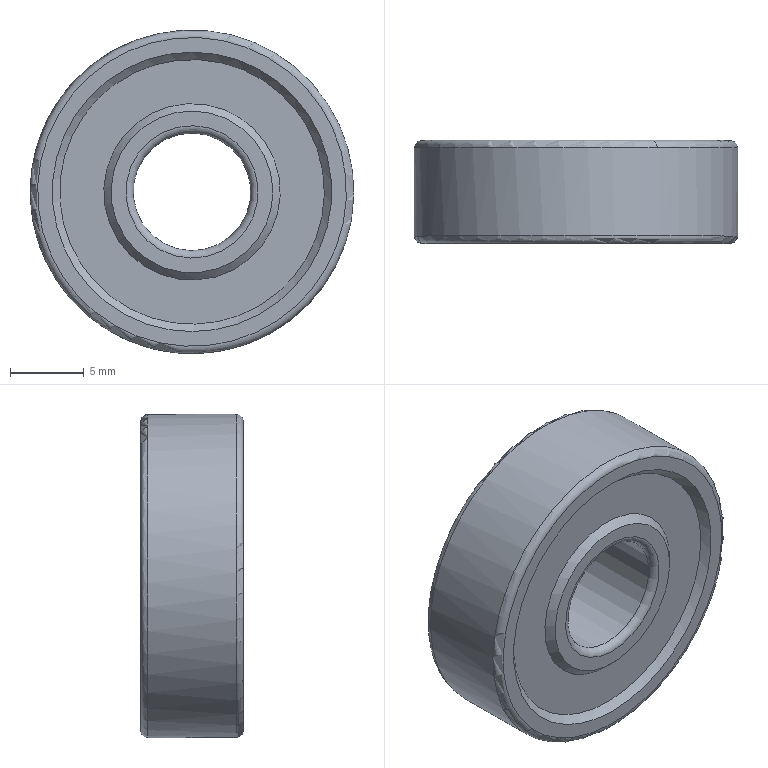Component | NX | BEARINGS | 1 solid | 16 faces | box 22 x 7 x 22 mm | volume 2134 mm3 | plane 6 | torus 4 | cone 4 | cylinder 2 | commonest cylinder face diameters 22 x1 8 x1
STEP:
#1=CARTESIAN_POINT('',(0.,0.,0.));
#2=DIRECTION('',(0.,0.,1.));
#3=DIRECTION('',(1.,0.,0.));
#4=AXIS2_PLACEMENT_3D('',#1,#2,#3);
#5=CARTESIAN_POINT('',(-426.878,103.5,-66.508));
#6=VERTEX_POINT('',#5);
#7=CARTESIAN_POINT('',(-422.274,103.5,-63.5));
#8=DIRECTION('',(0.,-1.,0.));
#9=DIRECTION('',(-0.8372,0.,-0.5469));
#10=AXIS2_PLACEMENT_3D('',#7,#8,#9);
#11=CIRCLE('',#10,5.5);
#12=CARTESIAN_POINT('',(-422.274,103.5,-63.5));
#13=DIRECTION('',(0.,-1.,0.));
#14=DIRECTION('',(-0.8372,0.,-0.5469));
#15=AXIS2_PLACEMENT_3D('',#12,#13,#14);
#16=PLANE('',#15);
#17=CARTESIAN_POINT('',(0.,0.));
#18=DIRECTION('',(1.,-0.));
#19=AXIS2_PLACEMENT_2D('',#17,#18);
#20=CIRCLE('',#19,5.5);
#21=(GEOMETRIC_REPRESENTATION_CONTEXT(2)PARAMETRIC_REPRESENTATION_CONTEXT()REPRESENTATION_CONTEXT('',''));
#22=DEFINITIONAL_REPRESENTATION('',(#20),#21);
#23=PCURVE('',#16,#22);
#24=CARTESIAN_POINT('',(-422.274,103.5,-63.5));
#25=DIRECTION('',(0.,1.,0.));
#26=DIRECTION('',(0.8372,0.,0.5469));
#27=AXIS2_PLACEMENT_3D('',#24,#25,#26);
#28=CONICAL_SURFACE('',#27,5.5,0.7854);
#29=CARTESIAN_POINT('',(9.425,0.));
#30=DIRECTION('',(-1.,0.));
#31=VECTOR('',#30,1.);
#32=LINE('',#29,#31);
#33=(GEOMETRIC_REPRESENTATION_CONTEXT(2)PARAMETRIC_REPRESENTATION_CONTEXT()REPRESENTATION_CONTEXT('',''));
#34=DEFINITIONAL_REPRESENTATION('',(#32),#33);
#35=PCURVE('',#28,#34);
#36=SURFACE_CURVE('',#11,(#23,#35),.PCURVE_S1.);
#37=EDGE_CURVE('',#6,#6,#36,.T.);
#38=ORIENTED_EDGE('',*,*,#37,.T.);
#39=EDGE_LOOP('',(#38));
#40=FACE_BOUND('',#39,.T.);
#41=CARTESIAN_POINT('',(-426.041,103.5,-65.961));
#42=VERTEX_POINT('',#41);
#43=CARTESIAN_POINT('',(-422.274,103.5,-63.5));
#44=DIRECTION('',(0.,1.,0.));
#45=DIRECTION('',(-0.8372,0.,-0.5469));
#46=AXIS2_PLACEMENT_3D('',#43,#44,#45);
#47=CIRCLE('',#46,4.5);
#48=CARTESIAN_POINT('',(4.5,0.));
#49=CARTESIAN_POINT('',(4.5,-7.794));
#50=CARTESIAN_POINT('',(-2.25,-3.897));
#51=CARTESIAN_POINT('',(-9.,-0.));
#52=CARTESIAN_POINT('',(-2.25,3.897));
#53=CARTESIAN_POINT('',(4.5,7.794));
#54=CARTESIAN_POINT('',(4.5,0.));
#55=(BOUNDED_CURVE()B_SPLINE_CURVE(2,(#48,#49,#50,#51,#52,#53,#54),.UNSPECIFIED.,.T.,.F.)B_SPLINE_CURVE_WITH_KNOTS((1,2,2,2,2,1),(-2.094,0.,2.094,4.189,6.283,8.378),.UNSPECIFIED.)CURVE()GEOMETRIC_REPRESENTATION_ITEM()RATIONAL_B_SPLINE_CURVE((1.,0.5,1.,0.5,1.,0.5,1.))REPRESENTATION_ITEM(''));
#56=(GEOMETRIC_REPRESENTATION_CONTEXT(2)PARAMETRIC_REPRESENTATION_CONTEXT()REPRESENTATION_CONTEXT('',''));
#57=DEFINITIONAL_REPRESENTATION('',(#55),#56);
#58=PCURVE('',#16,#57);
#59=CARTESIAN_POINT('',(-422.274,104.,-63.5));
#60=DIRECTION('',(0.,-1.,0.));
#61=DIRECTION('',(-0.8372,0.,-0.5469));
#62=AXIS2_PLACEMENT_3D('',#59,#60,#61);
#63=TOROIDAL_SURFACE('',#62,4.5,0.5);
#64=CARTESIAN_POINT('',(6.283,7.854));
#65=DIRECTION('',(-1.,0.));
#66=VECTOR('',#65,1.);
#67=LINE('',#64,#66);
#68=(GEOMETRIC_REPRESENTATION_CONTEXT(2)PARAMETRIC_REPRESENTATION_CONTEXT()REPRESENTATION_CONTEXT('',''));
#69=DEFINITIONAL_REPRESENTATION('',(#67),#68);
#70=PCURVE('',#63,#69);
#71=SURFACE_CURVE('',#47,(#58,#70),.PCURVE_S1.);
#72=EDGE_CURVE('',#42,#42,#71,.T.);
#73=ORIENTED_EDGE('',*,*,#72,.T.);
#74=EDGE_LOOP('',(#73));
#75=FACE_BOUND('',#74,.T.);
#76=ADVANCED_FACE('',(#40,#75),#16,.T.);
#77=CARTESIAN_POINT('',(-418.506,110.5,-61.039));
#78=VERTEX_POINT('',#77);
#79=CARTESIAN_POINT('',(-422.274,110.5,-63.5));
#80=DIRECTION('',(0.,-1.,0.));
#81=DIRECTION('',(0.8372,0.,0.5469));
#82=AXIS2_PLACEMENT_3D('',#79,#80,#81);
#83=CIRCLE('',#82,4.5);
#84=CARTESIAN_POINT('',(-422.274,110.5,-63.5));
#85=DIRECTION('',(0.,1.,0.));
#86=DIRECTION('',(0.8372,0.,0.5469));
#87=AXIS2_PLACEMENT_3D('',#84,#85,#86);
#88=PLANE('',#87);
#89=CARTESIAN_POINT('',(4.5,-0.));
#90=CARTESIAN_POINT('',(4.5,-7.794));
#91=CARTESIAN_POINT('',(-2.25,-3.897));
#92=CARTESIAN_POINT('',(-9.,0.));
#93=CARTESIAN_POINT('',(-2.25,3.897));
#94=CARTESIAN_POINT('',(4.5,7.794));
#95=CARTESIAN_POINT('',(4.5,-0.));
#96=(BOUNDED_CURVE()B_SPLINE_CURVE(2,(#89,#90,#91,#92,#93,#94,#95),.UNSPECIFIED.,.T.,.F.)B_SPLINE_CURVE_WITH_KNOTS((1,2,2,2,2,1),(-2.094,0.,2.094,4.189,6.283,8.378),.UNSPECIFIED.)CURVE()GEOMETRIC_REPRESENTATION_ITEM()RATIONAL_B_SPLINE_CURVE((1.,0.5,1.,0.5,1.,0.5,1.))REPRESENTATION_ITEM(''));
#97=(GEOMETRIC_REPRESENTATION_CONTEXT(2)PARAMETRIC_REPRESENTATION_CONTEXT()REPRESENTATION_CONTEXT('',''));
#98=DEFINITIONAL_REPRESENTATION('',(#96),#97);
#99=PCURVE('',#88,#98);
#100=CARTESIAN_POINT('',(-422.274,110.,-63.5));
#101=DIRECTION('',(0.,1.,0.));
#102=DIRECTION('',(0.8372,0.,0.5469));
#103=AXIS2_PLACEMENT_3D('',#100,#101,#102);
#104=TOROIDAL_SURFACE('',#103,4.5,0.5);
#105=CARTESIAN_POINT('',(6.283,7.854));
#106=DIRECTION('',(-1.,0.));
#107=VECTOR('',#106,1.);
#108=LINE('',#105,#107);
#109=(GEOMETRIC_REPRESENTATION_CONTEXT(2)PARAMETRIC_REPRESENTATION_CONTEXT()REPRESENTATION_CONTEXT('',''));
#110=DEFINITIONAL_REPRESENTATION('',(#108),#109);
#111=PCURVE('',#104,#110);
#112=SURFACE_CURVE('',#83,(#99,#111),.PCURVE_S1.);
#113=EDGE_CURVE('',#78,#78,#112,.T.);
#114=ORIENTED_EDGE('',*,*,#113,.T.);
#115=EDGE_LOOP('',(#114));
#116=FACE_BOUND('',#115,.T.);
#117=CARTESIAN_POINT('',(-417.669,110.5,-60.492));
#118=VERTEX_POINT('',#117);
#119=CARTESIAN_POINT('',(-422.274,110.5,-63.5));
#120=DIRECTION('',(0.,1.,0.));
#121=DIRECTION('',(0.8372,0.,0.5469));
#122=AXIS2_PLACEMENT_3D('',#119,#120,#121);
#123=CIRCLE('',#122,5.5);
#124=CARTESIAN_POINT('',(0.,0.));
#125=DIRECTION('',(1.,0.));
#126=AXIS2_PLACEMENT_2D('',#124,#125);
#127=CIRCLE('',#126,5.5);
#128=(GEOMETRIC_REPRESENTATION_CONTEXT(2)PARAMETRIC_REPRESENTATION_CONTEXT()REPRESENTATION_CONTEXT('',''));
#129=DEFINITIONAL_REPRESENTATION('',(#127),#128);
#130=PCURVE('',#88,#129);
#131=CARTESIAN_POINT('',(-422.274,110.,-63.5));
#132=DIRECTION('',(0.,-1.,0.));
#133=DIRECTION('',(-0.8372,0.,-0.5469));
#134=AXIS2_PLACEMENT_3D('',#131,#132,#133);
#135=CONICAL_SURFACE('',#134,6.,0.7854);
#136=CARTESIAN_POINT('',(9.425,-0.5));
#137=DIRECTION('',(-1.,0.));
#138=VECTOR('',#137,1.);
#139=LINE('',#136,#138);
#140=(GEOMETRIC_REPRESENTATION_CONTEXT(2)PARAMETRIC_REPRESENTATION_CONTEXT()REPRESENTATION_CONTEXT('',''));
#141=DEFINITIONAL_REPRESENTATION('',(#139),#140);
#142=PCURVE('',#135,#141);
#143=SURFACE_CURVE('',#123,(#130,#142),.PCURVE_S1.);
#144=EDGE_CURVE('',#118,#118,#143,.T.);
#145=ORIENTED_EDGE('',*,*,#144,.T.);
#146=EDGE_LOOP('',(#145));
#147=FACE_BOUND('',#146,.T.);
#148=ADVANCED_FACE('',(#116,#147),#88,.T.);
#149=CARTESIAN_POINT('',(-414.32,110.5,-58.304));
#150=VERTEX_POINT('',#149);
#151=CARTESIAN_POINT('',(-422.274,110.5,-63.5));
#152=DIRECTION('',(0.,1.,0.));
#153=DIRECTION('',(0.8372,0.,0.5469));
#154=AXIS2_PLACEMENT_3D('',#151,#152,#153);
#155=CIRCLE('',#154,9.5);
#156=CARTESIAN_POINT('',(-422.274,110.5,-63.5));
#157=DIRECTION('',(0.,1.,0.));
#158=DIRECTION('',(0.8372,0.,0.5469));
#159=AXIS2_PLACEMENT_3D('',#156,#157,#158);
#160=PLANE('',#159);
#161=CARTESIAN_POINT('',(0.,0.));
#162=DIRECTION('',(1.,0.));
#163=AXIS2_PLACEMENT_2D('',#161,#162);
#164=CIRCLE('',#163,9.5);
#165=(GEOMETRIC_REPRESENTATION_CONTEXT(2)PARAMETRIC_REPRESENTATION_CONTEXT()REPRESENTATION_CONTEXT('',''));
#166=DEFINITIONAL_REPRESENTATION('',(#164),#165);
#167=PCURVE('',#160,#166);
#168=CARTESIAN_POINT('',(-422.274,110.5,-63.5));
#169=DIRECTION('',(0.,1.,0.));
#170=DIRECTION('',(0.8372,0.,0.5469));
#171=AXIS2_PLACEMENT_3D('',#168,#169,#170);
#172=CONICAL_SURFACE('',#171,9.5,0.7854);
#173=CARTESIAN_POINT('',(0.,0.));
#174=DIRECTION('',(1.,0.));
#175=VECTOR('',#174,1.);
#176=LINE('',#173,#175);
#177=(GEOMETRIC_REPRESENTATION_CONTEXT(2)PARAMETRIC_REPRESENTATION_CONTEXT()REPRESENTATION_CONTEXT('',''));
#178=DEFINITIONAL_REPRESENTATION('',(#176),#177);
#179=PCURVE('',#172,#178);
#180=SURFACE_CURVE('',#155,(#167,#179),.PCURVE_S1.);
#181=EDGE_CURVE('',#150,#150,#180,.T.);
#182=ORIENTED_EDGE('',*,*,#181,.F.);
#183=EDGE_LOOP('',(#182));
#184=FACE_BOUND('',#183,.T.);
#185=CARTESIAN_POINT('',(-413.483,110.5,-57.757));
#186=VERTEX_POINT('',#185);
#187=CARTESIAN_POINT('',(-422.274,110.5,-63.5));
#188=DIRECTION('',(0.,1.,0.));
#189=DIRECTION('',(0.8372,0.,0.5469));
#190=AXIS2_PLACEMENT_3D('',#187,#188,#189);
#191=CIRCLE('',#190,10.5);
#192=CARTESIAN_POINT('',(0.,0.));
#193=DIRECTION('',(1.,0.));
#194=AXIS2_PLACEMENT_2D('',#192,#193);
#195=CIRCLE('',#194,10.5);
#196=(GEOMETRIC_REPRESENTATION_CONTEXT(2)PARAMETRIC_REPRESENTATION_CONTEXT()REPRESENTATION_CONTEXT('',''));
#197=DEFINITIONAL_REPRESENTATION('',(#195),#196);
#198=PCURVE('',#160,#197);
#199=CARTESIAN_POINT('',(-422.274,110.,-63.5));
#200=DIRECTION('',(0.,1.,0.));
#201=DIRECTION('',(0.8372,0.,0.5469));
#202=AXIS2_PLACEMENT_3D('',#199,#200,#201);
#203=TOROIDAL_SURFACE('',#202,10.5,0.5);
#204=CARTESIAN_POINT('',(0.,7.854));
#205=DIRECTION('',(1.,0.));
#206=VECTOR('',#205,1.);
#207=LINE('',#204,#206);
#208=(GEOMETRIC_REPRESENTATION_CONTEXT(2)PARAMETRIC_REPRESENTATION_CONTEXT()REPRESENTATION_CONTEXT('',''));
#209=DEFINITIONAL_REPRESENTATION('',(#207),#208);
#210=PCURVE('',#203,#209);
#211=SURFACE_CURVE('',#191,(#198,#210),.PCURVE_S1.);
#212=EDGE_CURVE('',#186,#186,#211,.T.);
#213=ORIENTED_EDGE('',*,*,#212,.T.);
#214=EDGE_LOOP('',(#213));
#215=FACE_BOUND('',#214,.T.);
#216=ADVANCED_FACE('',(#184,#215),#160,.T.);
#217=CARTESIAN_POINT('',(-430.227,103.5,-68.696));
#218=VERTEX_POINT('',#217);
#219=CARTESIAN_POINT('',(-422.274,103.5,-63.5));
#220=DIRECTION('',(0.,1.,0.));
#221=DIRECTION('',(-0.8372,0.,-0.5469));
#222=AXIS2_PLACEMENT_3D('',#219,#220,#221);
#223=CIRCLE('',#222,9.5);
#224=CARTESIAN_POINT('',(-422.274,103.5,-63.5));
#225=DIRECTION('',(0.,-1.,0.));
#226=DIRECTION('',(-0.8372,0.,-0.5469));
#227=AXIS2_PLACEMENT_3D('',#224,#225,#226);
#228=PLANE('',#227);
#229=CARTESIAN_POINT('',(9.5,0.));
#230=CARTESIAN_POINT('',(9.5,-16.454));
#231=CARTESIAN_POINT('',(-4.75,-8.227));
#232=CARTESIAN_POINT('',(-19.,-0.));
#233=CARTESIAN_POINT('',(-4.75,8.227));
#234=CARTESIAN_POINT('',(9.5,16.454));
#235=CARTESIAN_POINT('',(9.5,0.));
#236=(BOUNDED_CURVE()B_SPLINE_CURVE(2,(#229,#230,#231,#232,#233,#234,#235),.UNSPECIFIED.,.T.,.F.)B_SPLINE_CURVE_WITH_KNOTS((1,2,2,2,2,1),(-2.094,0.,2.094,4.189,6.283,8.378),.UNSPECIFIED.)CURVE()GEOMETRIC_REPRESENTATION_ITEM()RATIONAL_B_SPLINE_CURVE((1.,0.5,1.,0.5,1.,0.5,1.))REPRESENTATION_ITEM(''));
#237=(GEOMETRIC_REPRESENTATION_CONTEXT(2)PARAMETRIC_REPRESENTATION_CONTEXT()REPRESENTATION_CONTEXT('',''));
#238=DEFINITIONAL_REPRESENTATION('',(#236),#237);
#239=PCURVE('',#228,#238);
#240=CARTESIAN_POINT('',(-422.274,103.5,-63.5));
#241=DIRECTION('',(0.,-1.,0.));
#242=DIRECTION('',(-0.8372,0.,-0.5469));
#243=AXIS2_PLACEMENT_3D('',#240,#241,#242);
#244=CONICAL_SURFACE('',#243,9.5,0.7854);
#245=CARTESIAN_POINT('',(6.283,0.));
#246=DIRECTION('',(-1.,0.));
#247=VECTOR('',#246,1.);
#248=LINE('',#245,#247);
#249=(GEOMETRIC_REPRESENTATION_CONTEXT(2)PARAMETRIC_REPRESENTATION_CONTEXT()REPRESENTATION_CONTEXT('',''));
#250=DEFINITIONAL_REPRESENTATION('',(#248),#249);
#251=PCURVE('',#244,#250);
#252=SURFACE_CURVE('',#223,(#239,#251),.PCURVE_S1.);
#253=EDGE_CURVE('',#218,#218,#252,.T.);
#254=ORIENTED_EDGE('',*,*,#253,.T.);
#255=EDGE_LOOP('',(#254));
#256=FACE_BOUND('',#255,.T.);
#257=CARTESIAN_POINT('',(-431.064,103.5,-69.243));
#258=VERTEX_POINT('',#257);
#259=CARTESIAN_POINT('',(-422.274,103.5,-63.5));
#260=DIRECTION('',(0.,-1.,0.));
#261=DIRECTION('',(-0.8372,0.,-0.5469));
#262=AXIS2_PLACEMENT_3D('',#259,#260,#261);
#263=CIRCLE('',#262,10.5);
#264=CARTESIAN_POINT('',(0.,0.));
#265=DIRECTION('',(1.,-0.));
#266=AXIS2_PLACEMENT_2D('',#264,#265);
#267=CIRCLE('',#266,10.5);
#268=(GEOMETRIC_REPRESENTATION_CONTEXT(2)PARAMETRIC_REPRESENTATION_CONTEXT()REPRESENTATION_CONTEXT('',''));
#269=DEFINITIONAL_REPRESENTATION('',(#267),#268);
#270=PCURVE('',#228,#269);
#271=CARTESIAN_POINT('',(-422.274,104.,-63.5));
#272=DIRECTION('',(0.,-1.,0.));
#273=DIRECTION('',(-0.8372,0.,-0.5469));
#274=AXIS2_PLACEMENT_3D('',#271,#272,#273);
#275=TOROIDAL_SURFACE('',#274,10.5,0.5);
#276=CARTESIAN_POINT('',(0.,7.854));
#277=DIRECTION('',(1.,0.));
#278=VECTOR('',#277,1.);
#279=LINE('',#276,#278);
#280=(GEOMETRIC_REPRESENTATION_CONTEXT(2)PARAMETRIC_REPRESENTATION_CONTEXT()REPRESENTATION_CONTEXT('',''));
#281=DEFINITIONAL_REPRESENTATION('',(#279),#280);
#282=PCURVE('',#275,#281);
#283=SURFACE_CURVE('',#263,(#270,#282),.PCURVE_S1.);
#284=EDGE_CURVE('',#258,#258,#283,.T.);
#285=ORIENTED_EDGE('',*,*,#284,.T.);
#286=EDGE_LOOP('',(#285));
#287=FACE_BOUND('',#286,.T.);
#288=ADVANCED_FACE('',(#256,#287),#228,.T.);
#289=CARTESIAN_POINT('',(-431.482,104.,-69.516));
#290=VERTEX_POINT('',#289);
#291=CARTESIAN_POINT('',(-413.065,104.,-57.484));
#292=VERTEX_POINT('',#291);
#293=CARTESIAN_POINT('',(-422.274,104.,-63.5));
#294=DIRECTION('',(0.,1.,0.));
#295=DIRECTION('',(-0.8372,0.,-0.5469));
#296=AXIS2_PLACEMENT_3D('',#293,#294,#295);
#297=CIRCLE('',#296,11.);
#298=CARTESIAN_POINT('',(-422.274,103.5,-63.5));
#299=DIRECTION('',(0.,1.,0.));
#300=DIRECTION('',(0.8372,0.,0.5469));
#301=AXIS2_PLACEMENT_3D('',#298,#299,#300);
#302=CYLINDRICAL_SURFACE('',#301,11.);
#303=CARTESIAN_POINT('',(3.142,0.5));
#304=DIRECTION('',(1.,0.));
#305=VECTOR('',#304,1.);
#306=LINE('',#303,#305);
#307=(GEOMETRIC_REPRESENTATION_CONTEXT(2)PARAMETRIC_REPRESENTATION_CONTEXT()REPRESENTATION_CONTEXT('',''));
#308=DEFINITIONAL_REPRESENTATION('',(#306),#307);
#309=PCURVE('',#302,#308);
#310=CARTESIAN_POINT('',(6.283,6.283));
#311=DIRECTION('',(-1.,0.));
#312=VECTOR('',#311,1.);
#313=LINE('',#310,#312);
#314=(GEOMETRIC_REPRESENTATION_CONTEXT(2)PARAMETRIC_REPRESENTATION_CONTEXT()REPRESENTATION_CONTEXT('',''));
#315=DEFINITIONAL_REPRESENTATION('',(#313),#314);
#316=PCURVE('',#275,#315);
#317=SURFACE_CURVE('',#297,(#309,#316),.PCURVE_S1.);
#318=EDGE_CURVE('',#290,#292,#317,.T.);
#319=ORIENTED_EDGE('',*,*,#318,.T.);
#320=CARTESIAN_POINT('',(-413.065,110.,-57.484));
#321=VERTEX_POINT('',#320);
#322=CARTESIAN_POINT('',(-413.065,104.,-57.484));
#323=CARTESIAN_POINT('',(-413.065,110.,-57.484));
#324=B_SPLINE_CURVE_WITH_KNOTS('',1,(#322,#323),.UNSPECIFIED.,.F.,.F.,(2,2),(0.5,6.5),.PIECEWISE_BEZIER_KNOTS.);
#325=CARTESIAN_POINT('',(6.283,0.));
#326=DIRECTION('',(0.,1.));
#327=VECTOR('',#326,1.);
#328=LINE('',#325,#327);
#329=(GEOMETRIC_REPRESENTATION_CONTEXT(2)PARAMETRIC_REPRESENTATION_CONTEXT()REPRESENTATION_CONTEXT('',''));
#330=DEFINITIONAL_REPRESENTATION('',(#328),#329);
#331=PCURVE('',#302,#330);
#332=CARTESIAN_POINT('',(0.,0.));
#333=DIRECTION('',(0.,1.));
#334=VECTOR('',#333,1.);
#335=LINE('',#332,#334);
#336=(GEOMETRIC_REPRESENTATION_CONTEXT(2)PARAMETRIC_REPRESENTATION_CONTEXT()REPRESENTATION_CONTEXT('',''));
#337=DEFINITIONAL_REPRESENTATION('',(#335),#336);
#338=PCURVE('',#302,#337);
#339=SEAM_CURVE('',#324,(#331,#338),.PCURVE_S1.);
#340=EDGE_CURVE('',#292,#321,#339,.T.);
#341=ORIENTED_EDGE('',*,*,#340,.T.);
#342=CARTESIAN_POINT('',(-422.274,110.,-63.5));
#343=DIRECTION('',(0.,-1.,0.));
#344=DIRECTION('',(0.8372,0.,0.5469));
#345=AXIS2_PLACEMENT_3D('',#342,#343,#344);
#346=CIRCLE('',#345,11.);
#347=CARTESIAN_POINT('',(6.283,6.5));
#348=DIRECTION('',(-1.,0.));
#349=VECTOR('',#348,1.);
#350=LINE('',#347,#349);
#351=(GEOMETRIC_REPRESENTATION_CONTEXT(2)PARAMETRIC_REPRESENTATION_CONTEXT()REPRESENTATION_CONTEXT('',''));
#352=DEFINITIONAL_REPRESENTATION('',(#350),#351);
#353=PCURVE('',#302,#352);
#354=CARTESIAN_POINT('',(6.283,6.283));
#355=DIRECTION('',(-1.,0.));
#356=VECTOR('',#355,1.);
#357=LINE('',#354,#356);
#358=(GEOMETRIC_REPRESENTATION_CONTEXT(2)PARAMETRIC_REPRESENTATION_CONTEXT()REPRESENTATION_CONTEXT('',''));
#359=DEFINITIONAL_REPRESENTATION('',(#357),#358);
#360=PCURVE('',#203,#359);
#361=SURFACE_CURVE('',#346,(#353,#360),.PCURVE_S1.);
#362=EDGE_CURVE('',#321,#321,#361,.T.);
#363=ORIENTED_EDGE('',*,*,#362,.T.);
#364=ORIENTED_EDGE('',*,*,#340,.F.);
#365=CARTESIAN_POINT('',(-422.274,104.,-63.5));
#366=DIRECTION('',(0.,1.,0.));
#367=DIRECTION('',(-0.8372,0.,-0.5469));
#368=AXIS2_PLACEMENT_3D('',#365,#366,#367);
#369=CIRCLE('',#368,11.);
#370=CARTESIAN_POINT('',(-3.142,0.5));
#371=DIRECTION('',(1.,0.));
#372=VECTOR('',#371,1.);
#373=LINE('',#370,#372);
#374=(GEOMETRIC_REPRESENTATION_CONTEXT(2)PARAMETRIC_REPRESENTATION_CONTEXT()REPRESENTATION_CONTEXT('',''));
#375=DEFINITIONAL_REPRESENTATION('',(#373),#374);
#376=PCURVE('',#302,#375);
#377=CARTESIAN_POINT('',(6.283,6.283));
#378=DIRECTION('',(-1.,0.));
#379=VECTOR('',#378,1.);
#380=LINE('',#377,#379);
#381=(GEOMETRIC_REPRESENTATION_CONTEXT(2)PARAMETRIC_REPRESENTATION_CONTEXT()REPRESENTATION_CONTEXT('',''));
#382=DEFINITIONAL_REPRESENTATION('',(#380),#381);
#383=PCURVE('',#275,#382);
#384=SURFACE_CURVE('',#369,(#376,#383),.PCURVE_S1.);
#385=EDGE_CURVE('',#292,#290,#384,.T.);
#386=ORIENTED_EDGE('',*,*,#385,.T.);
#387=EDGE_LOOP('',(#319,#341,#363,#364,#386));
#388=FACE_BOUND('',#387,.T.);
#389=ADVANCED_FACE('',(#388),#302,.T.);
#390=CARTESIAN_POINT('',(-418.925,104.,-61.312));
#391=VERTEX_POINT('',#390);
#392=CARTESIAN_POINT('',(-425.622,104.,-65.688));
#393=VERTEX_POINT('',#392);
#394=CARTESIAN_POINT('',(-422.274,104.,-63.5));
#395=DIRECTION('',(0.,-1.,0.));
#396=DIRECTION('',(-0.8372,0.,-0.5469));
#397=AXIS2_PLACEMENT_3D('',#394,#395,#396);
#398=CIRCLE('',#397,4.);
#399=CARTESIAN_POINT('',(-422.274,110.5,-63.5));
#400=DIRECTION('',(0.,-1.,0.));
#401=DIRECTION('',(0.8372,0.,0.5469));
#402=AXIS2_PLACEMENT_3D('',#399,#400,#401);
#403=CYLINDRICAL_SURFACE('',#402,4.);
#404=CARTESIAN_POINT('',(-3.142,6.5));
#405=DIRECTION('',(1.,0.));
#406=VECTOR('',#405,1.);
#407=LINE('',#404,#406);
#408=(GEOMETRIC_REPRESENTATION_CONTEXT(2)PARAMETRIC_REPRESENTATION_CONTEXT()REPRESENTATION_CONTEXT('',''));
#409=DEFINITIONAL_REPRESENTATION('',(#407),#408);
#410=PCURVE('',#403,#409);
#411=CARTESIAN_POINT('',(0.,9.425));
#412=DIRECTION('',(1.,0.));
#413=VECTOR('',#412,1.);
#414=LINE('',#411,#413);
#415=(GEOMETRIC_REPRESENTATION_CONTEXT(2)PARAMETRIC_REPRESENTATION_CONTEXT()REPRESENTATION_CONTEXT('',''));
#416=DEFINITIONAL_REPRESENTATION('',(#414),#415);
#417=PCURVE('',#63,#416);
#418=SURFACE_CURVE('',#398,(#410,#417),.PCURVE_S1.);
#419=EDGE_CURVE('',#391,#393,#418,.T.);
#420=ORIENTED_EDGE('',*,*,#419,.F.);
#421=CARTESIAN_POINT('',(-418.925,110.,-61.312));
#422=VERTEX_POINT('',#421);
#423=CARTESIAN_POINT('',(-418.925,110.,-61.312));
#424=CARTESIAN_POINT('',(-418.925,104.,-61.312));
#425=B_SPLINE_CURVE_WITH_KNOTS('',1,(#423,#424),.UNSPECIFIED.,.F.,.F.,(2,2),(0.5,6.5),.PIECEWISE_BEZIER_KNOTS.);
#426=CARTESIAN_POINT('',(0.,0.));
#427=DIRECTION('',(0.,1.));
#428=VECTOR('',#427,1.);
#429=LINE('',#426,#428);
#430=(GEOMETRIC_REPRESENTATION_CONTEXT(2)PARAMETRIC_REPRESENTATION_CONTEXT()REPRESENTATION_CONTEXT('',''));
#431=DEFINITIONAL_REPRESENTATION('',(#429),#430);
#432=PCURVE('',#403,#431);
#433=CARTESIAN_POINT('',(6.283,0.));
#434=DIRECTION('',(0.,1.));
#435=VECTOR('',#434,1.);
#436=LINE('',#433,#435);
#437=(GEOMETRIC_REPRESENTATION_CONTEXT(2)PARAMETRIC_REPRESENTATION_CONTEXT()REPRESENTATION_CONTEXT('',''));
#438=DEFINITIONAL_REPRESENTATION('',(#436),#437);
#439=PCURVE('',#403,#438);
#440=SEAM_CURVE('',#425,(#432,#439),.PCURVE_S1.);
#441=EDGE_CURVE('',#422,#391,#440,.T.);
#442=ORIENTED_EDGE('',*,*,#441,.F.);
#443=CARTESIAN_POINT('',(-422.274,110.,-63.5));
#444=DIRECTION('',(0.,1.,0.));
#445=DIRECTION('',(0.8372,0.,0.5469));
#446=AXIS2_PLACEMENT_3D('',#443,#444,#445);
#447=CIRCLE('',#446,4.);
#448=CARTESIAN_POINT('',(6.283,0.5));
#449=DIRECTION('',(-1.,0.));
#450=VECTOR('',#449,1.);
#451=LINE('',#448,#450);
#452=(GEOMETRIC_REPRESENTATION_CONTEXT(2)PARAMETRIC_REPRESENTATION_CONTEXT()REPRESENTATION_CONTEXT('',''));
#453=DEFINITIONAL_REPRESENTATION('',(#451),#452);
#454=PCURVE('',#403,#453);
#455=CARTESIAN_POINT('',(0.,9.425));
#456=DIRECTION('',(1.,0.));
#457=VECTOR('',#456,1.);
#458=LINE('',#455,#457);
#459=(GEOMETRIC_REPRESENTATION_CONTEXT(2)PARAMETRIC_REPRESENTATION_CONTEXT()REPRESENTATION_CONTEXT('',''));
#460=DEFINITIONAL_REPRESENTATION('',(#458),#459);
#461=PCURVE('',#104,#460);
#462=SURFACE_CURVE('',#447,(#454,#461),.PCURVE_S1.);
#463=EDGE_CURVE('',#422,#422,#462,.T.);
#464=ORIENTED_EDGE('',*,*,#463,.F.);
#465=ORIENTED_EDGE('',*,*,#441,.T.);
#466=CARTESIAN_POINT('',(-422.274,104.,-63.5));
#467=DIRECTION('',(0.,-1.,0.));
#468=DIRECTION('',(-0.8372,0.,-0.5469));
#469=AXIS2_PLACEMENT_3D('',#466,#467,#468);
#470=CIRCLE('',#469,4.);
#471=CARTESIAN_POINT('',(3.142,6.5));
#472=DIRECTION('',(1.,0.));
#473=VECTOR('',#472,1.);
#474=LINE('',#471,#473);
#475=(GEOMETRIC_REPRESENTATION_CONTEXT(2)PARAMETRIC_REPRESENTATION_CONTEXT()REPRESENTATION_CONTEXT('',''));
#476=DEFINITIONAL_REPRESENTATION('',(#474),#475);
#477=PCURVE('',#403,#476);
#478=CARTESIAN_POINT('',(0.,9.425));
#479=DIRECTION('',(1.,-0.));
#480=VECTOR('',#479,1.);
#481=LINE('',#478,#480);
#482=(GEOMETRIC_REPRESENTATION_CONTEXT(2)PARAMETRIC_REPRESENTATION_CONTEXT()REPRESENTATION_CONTEXT('',''));
#483=DEFINITIONAL_REPRESENTATION('',(#481),#482);
#484=PCURVE('',#63,#483);
#485=SURFACE_CURVE('',#470,(#477,#484),.PCURVE_S1.);
#486=EDGE_CURVE('',#393,#391,#485,.T.);
#487=ORIENTED_EDGE('',*,*,#486,.F.);
#488=EDGE_LOOP('',(#420,#442,#464,#465,#487));
#489=FACE_BOUND('',#488,.F.);
#490=ADVANCED_FACE('',(#489),#403,.F.);
#491=ORIENTED_EDGE('',*,*,#284,.F.);
#492=CARTESIAN_POINT('',(-431.482,104.,-69.516));
#493=CARTESIAN_POINT('',(-431.482,103.866,-69.516));
#494=CARTESIAN_POINT('',(-431.447,103.736,-69.493));
#495=CARTESIAN_POINT('',(-431.379,103.624,-69.449));
#496=CARTESIAN_POINT('',(-431.285,103.543,-69.387));
#497=CARTESIAN_POINT('',(-431.176,103.5,-69.316));
#498=CARTESIAN_POINT('',(-431.064,103.5,-69.243));
#499=(BOUNDED_CURVE()B_SPLINE_CURVE(6,(#492,#493,#494,#495,#496,#497,#498),.UNSPECIFIED.,.F.,.F.)B_SPLINE_CURVE_WITH_KNOTS((7,7),(0.,1.571),.PIECEWISE_BEZIER_KNOTS.)CURVE()GEOMETRIC_REPRESENTATION_ITEM()RATIONAL_B_SPLINE_CURVE((1.031,1.01,0.9979,0.994,0.9979,1.01,1.031))REPRESENTATION_ITEM(''));
#500=CARTESIAN_POINT('',(0.,6.283));
#501=DIRECTION('',(0.,1.));
#502=VECTOR('',#501,1.);
#503=LINE('',#500,#502);
#504=(GEOMETRIC_REPRESENTATION_CONTEXT(2)PARAMETRIC_REPRESENTATION_CONTEXT()REPRESENTATION_CONTEXT('',''));
#505=DEFINITIONAL_REPRESENTATION('',(#503),#504);
#506=PCURVE('',#275,#505);
#507=CARTESIAN_POINT('',(6.283,6.283));
#508=DIRECTION('',(0.,1.));
#509=VECTOR('',#508,1.);
#510=LINE('',#507,#509);
#511=(GEOMETRIC_REPRESENTATION_CONTEXT(2)PARAMETRIC_REPRESENTATION_CONTEXT()REPRESENTATION_CONTEXT('',''));
#512=DEFINITIONAL_REPRESENTATION('',(#510),#511);
#513=PCURVE('',#275,#512);
#514=SEAM_CURVE('',#499,(#506,#513),.PCURVE_S1.);
#515=EDGE_CURVE('',#290,#258,#514,.T.);
#516=ORIENTED_EDGE('',*,*,#515,.F.);
#517=ORIENTED_EDGE('',*,*,#385,.F.);
#518=ORIENTED_EDGE('',*,*,#318,.F.);
#519=ORIENTED_EDGE('',*,*,#515,.T.);
#520=EDGE_LOOP('',(#491,#516,#517,#518,#519));
#521=FACE_BOUND('',#520,.T.);
#522=ADVANCED_FACE('',(#521),#275,.T.);
#523=ORIENTED_EDGE('',*,*,#212,.F.);
#524=CARTESIAN_POINT('',(-413.065,110.,-57.484));
#525=CARTESIAN_POINT('',(-413.065,110.134,-57.484));
#526=CARTESIAN_POINT('',(-413.1,110.264,-57.507));
#527=CARTESIAN_POINT('',(-413.168,110.376,-57.551));
#528=CARTESIAN_POINT('',(-413.262,110.457,-57.613));
#529=CARTESIAN_POINT('',(-413.371,110.5,-57.684));
#530=CARTESIAN_POINT('',(-413.483,110.5,-57.757));
#531=(BOUNDED_CURVE()B_SPLINE_CURVE(6,(#524,#525,#526,#527,#528,#529,#530),.UNSPECIFIED.,.F.,.F.)B_SPLINE_CURVE_WITH_KNOTS((7,7),(0.,1.571),.PIECEWISE_BEZIER_KNOTS.)CURVE()GEOMETRIC_REPRESENTATION_ITEM()RATIONAL_B_SPLINE_CURVE((1.031,1.01,0.9979,0.994,0.9979,1.01,1.031))REPRESENTATION_ITEM(''));
#532=CARTESIAN_POINT('',(0.,6.283));
#533=DIRECTION('',(0.,1.));
#534=VECTOR('',#533,1.);
#535=LINE('',#532,#534);
#536=(GEOMETRIC_REPRESENTATION_CONTEXT(2)PARAMETRIC_REPRESENTATION_CONTEXT()REPRESENTATION_CONTEXT('',''));
#537=DEFINITIONAL_REPRESENTATION('',(#535),#536);
#538=PCURVE('',#203,#537);
#539=CARTESIAN_POINT('',(6.283,6.283));
#540=DIRECTION('',(0.,1.));
#541=VECTOR('',#540,1.);
#542=LINE('',#539,#541);
#543=(GEOMETRIC_REPRESENTATION_CONTEXT(2)PARAMETRIC_REPRESENTATION_CONTEXT()REPRESENTATION_CONTEXT('',''));
#544=DEFINITIONAL_REPRESENTATION('',(#542),#543);
#545=PCURVE('',#203,#544);
#546=SEAM_CURVE('',#531,(#538,#545),.PCURVE_S1.);
#547=EDGE_CURVE('',#321,#186,#546,.T.);
#548=ORIENTED_EDGE('',*,*,#547,.F.);
#549=ORIENTED_EDGE('',*,*,#362,.F.);
#550=ORIENTED_EDGE('',*,*,#547,.T.);
#551=EDGE_LOOP('',(#523,#548,#549,#550));
#552=FACE_BOUND('',#551,.T.);
#553=ADVANCED_FACE('',(#552),#203,.T.);
#554=ORIENTED_EDGE('',*,*,#486,.F.);
#555=CARTESIAN_POINT('',(-426.041,103.5,-65.961));
#556=CARTESIAN_POINT('',(-425.929,103.5,-65.888));
#557=CARTESIAN_POINT('',(-425.82,103.543,-65.817));
#558=CARTESIAN_POINT('',(-425.726,103.624,-65.756));
#559=CARTESIAN_POINT('',(-425.658,103.736,-65.711));
#560=CARTESIAN_POINT('',(-425.622,103.866,-65.688));
#561=CARTESIAN_POINT('',(-425.622,104.,-65.688));
#562=(BOUNDED_CURVE()B_SPLINE_CURVE(6,(#555,#556,#557,#558,#559,#560,#561),.UNSPECIFIED.,.F.,.F.)B_SPLINE_CURVE_WITH_KNOTS((7,7),(1.571,3.142),.PIECEWISE_BEZIER_KNOTS.)CURVE()GEOMETRIC_REPRESENTATION_ITEM()RATIONAL_B_SPLINE_CURVE((1.031,1.01,0.9979,0.994,0.9979,1.01,1.031))REPRESENTATION_ITEM(''));
#563=CARTESIAN_POINT('',(0.,6.283));
#564=DIRECTION('',(0.,1.));
#565=VECTOR('',#564,1.);
#566=LINE('',#563,#565);
#567=(GEOMETRIC_REPRESENTATION_CONTEXT(2)PARAMETRIC_REPRESENTATION_CONTEXT()REPRESENTATION_CONTEXT('',''));
#568=DEFINITIONAL_REPRESENTATION('',(#566),#567);
#569=PCURVE('',#63,#568);
#570=CARTESIAN_POINT('',(6.283,6.283));
#571=DIRECTION('',(0.,1.));
#572=VECTOR('',#571,1.);
#573=LINE('',#570,#572);
#574=(GEOMETRIC_REPRESENTATION_CONTEXT(2)PARAMETRIC_REPRESENTATION_CONTEXT()REPRESENTATION_CONTEXT('',''));
#575=DEFINITIONAL_REPRESENTATION('',(#573),#574);
#576=PCURVE('',#63,#575);
#577=SEAM_CURVE('',#562,(#569,#576),.PCURVE_S1.);
#578=EDGE_CURVE('',#42,#393,#577,.T.);
#579=ORIENTED_EDGE('',*,*,#578,.F.);
#580=ORIENTED_EDGE('',*,*,#72,.F.);
#581=ORIENTED_EDGE('',*,*,#578,.T.);
#582=ORIENTED_EDGE('',*,*,#419,.F.);
#583=EDGE_LOOP('',(#554,#579,#580,#581,#582));
#584=FACE_BOUND('',#583,.T.);
#585=ADVANCED_FACE('',(#584),#63,.T.);
#586=ORIENTED_EDGE('',*,*,#463,.F.);
#587=CARTESIAN_POINT('',(-418.506,110.5,-61.039));
#588=CARTESIAN_POINT('',(-418.618,110.5,-61.112));
#589=CARTESIAN_POINT('',(-418.727,110.457,-61.183));
#590=CARTESIAN_POINT('',(-418.821,110.376,-61.244));
#591=CARTESIAN_POINT('',(-418.889,110.264,-61.289));
#592=CARTESIAN_POINT('',(-418.925,110.134,-61.312));
#593=CARTESIAN_POINT('',(-418.925,110.,-61.312));
#594=(BOUNDED_CURVE()B_SPLINE_CURVE(6,(#587,#588,#589,#590,#591,#592,#593),.UNSPECIFIED.,.F.,.F.)B_SPLINE_CURVE_WITH_KNOTS((7,7),(1.571,3.142),.PIECEWISE_BEZIER_KNOTS.)CURVE()GEOMETRIC_REPRESENTATION_ITEM()RATIONAL_B_SPLINE_CURVE((1.031,1.01,0.9979,0.994,0.9979,1.01,1.031))REPRESENTATION_ITEM(''));
#595=CARTESIAN_POINT('',(0.,6.283));
#596=DIRECTION('',(0.,1.));
#597=VECTOR('',#596,1.);
#598=LINE('',#595,#597);
#599=(GEOMETRIC_REPRESENTATION_CONTEXT(2)PARAMETRIC_REPRESENTATION_CONTEXT()REPRESENTATION_CONTEXT('',''));
#600=DEFINITIONAL_REPRESENTATION('',(#598),#599);
#601=PCURVE('',#104,#600);
#602=CARTESIAN_POINT('',(6.283,6.283));
#603=DIRECTION('',(0.,1.));
#604=VECTOR('',#603,1.);
#605=LINE('',#602,#604);
#606=(GEOMETRIC_REPRESENTATION_CONTEXT(2)PARAMETRIC_REPRESENTATION_CONTEXT()REPRESENTATION_CONTEXT('',''));
#607=DEFINITIONAL_REPRESENTATION('',(#605),#606);
#608=PCURVE('',#104,#607);
#609=SEAM_CURVE('',#594,(#601,#608),.PCURVE_S1.);
#610=EDGE_CURVE('',#78,#422,#609,.T.);
#611=ORIENTED_EDGE('',*,*,#610,.F.);
#612=ORIENTED_EDGE('',*,*,#113,.F.);
#613=ORIENTED_EDGE('',*,*,#610,.T.);
#614=EDGE_LOOP('',(#586,#611,#612,#613));
#615=FACE_BOUND('',#614,.T.);
#616=ADVANCED_FACE('',(#615),#104,.T.);
#617=CARTESIAN_POINT('',(-414.739,110.,-58.578));
#618=VERTEX_POINT('',#617);
#619=CARTESIAN_POINT('',(-422.274,110.,-63.5));
#620=DIRECTION('',(0.,1.,0.));
#621=DIRECTION('',(0.8372,0.,0.5469));
#622=AXIS2_PLACEMENT_3D('',#619,#620,#621);
#623=CIRCLE('',#622,9.);
#624=CARTESIAN_POINT('',(-422.274,110.,-63.5));
#625=DIRECTION('',(0.,1.,0.));
#626=DIRECTION('',(0.8372,0.,0.5469));
#627=AXIS2_PLACEMENT_3D('',#624,#625,#626);
#628=PLANE('',#627);
#629=CARTESIAN_POINT('',(0.,0.));
#630=DIRECTION('',(1.,0.));
#631=AXIS2_PLACEMENT_2D('',#629,#630);
#632=CIRCLE('',#631,9.);
#633=(GEOMETRIC_REPRESENTATION_CONTEXT(2)PARAMETRIC_REPRESENTATION_CONTEXT()REPRESENTATION_CONTEXT('',''));
#634=DEFINITIONAL_REPRESENTATION('',(#632),#633);
#635=PCURVE('',#628,#634);
#636=CARTESIAN_POINT('',(0.,-0.5));
#637=DIRECTION('',(1.,0.));
#638=VECTOR('',#637,1.);
#639=LINE('',#636,#638);
#640=(GEOMETRIC_REPRESENTATION_CONTEXT(2)PARAMETRIC_REPRESENTATION_CONTEXT()REPRESENTATION_CONTEXT('',''));
#641=DEFINITIONAL_REPRESENTATION('',(#639),#640);
#642=PCURVE('',#172,#641);
#643=SURFACE_CURVE('',#623,(#635,#642),.PCURVE_S1.);
#644=EDGE_CURVE('',#618,#618,#643,.T.);
#645=ORIENTED_EDGE('',*,*,#644,.T.);
#646=EDGE_LOOP('',(#645));
#647=FACE_BOUND('',#646,.T.);
#648=CARTESIAN_POINT('',(-417.251,110.,-60.218));
#649=VERTEX_POINT('',#648);
#650=CARTESIAN_POINT('',(-422.274,110.,-63.5));
#651=DIRECTION('',(0.,-1.,0.));
#652=DIRECTION('',(0.8372,0.,0.5469));
#653=AXIS2_PLACEMENT_3D('',#650,#651,#652);
#654=CIRCLE('',#653,6.);
#655=CARTESIAN_POINT('',(6.,-0.));
#656=CARTESIAN_POINT('',(6.,-10.392));
#657=CARTESIAN_POINT('',(-3.,-5.196));
#658=CARTESIAN_POINT('',(-12.,0.));
#659=CARTESIAN_POINT('',(-3.,5.196));
#660=CARTESIAN_POINT('',(6.,10.392));
#661=CARTESIAN_POINT('',(6.,-0.));
#662=(BOUNDED_CURVE()B_SPLINE_CURVE(2,(#655,#656,#657,#658,#659,#660,#661),.UNSPECIFIED.,.T.,.F.)B_SPLINE_CURVE_WITH_KNOTS((1,2,2,2,2,1),(-2.094,0.,2.094,4.189,6.283,8.378),.UNSPECIFIED.)CURVE()GEOMETRIC_REPRESENTATION_ITEM()RATIONAL_B_SPLINE_CURVE((1.,0.5,1.,0.5,1.,0.5,1.))REPRESENTATION_ITEM(''));
#663=(GEOMETRIC_REPRESENTATION_CONTEXT(2)PARAMETRIC_REPRESENTATION_CONTEXT()REPRESENTATION_CONTEXT('',''));
#664=DEFINITIONAL_REPRESENTATION('',(#662),#663);
#665=PCURVE('',#628,#664);
#666=CARTESIAN_POINT('',(3.142,0.));
#667=DIRECTION('',(1.,0.));
#668=VECTOR('',#667,1.);
#669=LINE('',#666,#668);
#670=(GEOMETRIC_REPRESENTATION_CONTEXT(2)PARAMETRIC_REPRESENTATION_CONTEXT()REPRESENTATION_CONTEXT('',''));
#671=DEFINITIONAL_REPRESENTATION('',(#669),#670);
#672=PCURVE('',#135,#671);
#673=SURFACE_CURVE('',#654,(#665,#672),.PCURVE_S1.);
#674=EDGE_CURVE('',#649,#649,#673,.T.);
#675=ORIENTED_EDGE('',*,*,#674,.T.);
#676=EDGE_LOOP('',(#675));
#677=FACE_BOUND('',#676,.T.);
#678=ADVANCED_FACE('',(#647,#677),#628,.T.);
#679=CARTESIAN_POINT('',(-427.297,104.,-66.782));
#680=VERTEX_POINT('',#679);
#681=CARTESIAN_POINT('',(-422.274,104.,-63.5));
#682=DIRECTION('',(0.,1.,0.));
#683=DIRECTION('',(-0.8372,0.,-0.5469));
#684=AXIS2_PLACEMENT_3D('',#681,#682,#683);
#685=CIRCLE('',#684,6.);
#686=CARTESIAN_POINT('',(-422.274,104.,-63.5));
#687=DIRECTION('',(0.,-1.,0.));
#688=DIRECTION('',(-0.8372,0.,-0.5469));
#689=AXIS2_PLACEMENT_3D('',#686,#687,#688);
#690=PLANE('',#689);
#691=CARTESIAN_POINT('',(6.,0.));
#692=CARTESIAN_POINT('',(6.,-10.392));
#693=CARTESIAN_POINT('',(-3.,-5.196));
#694=CARTESIAN_POINT('',(-12.,-0.));
#695=CARTESIAN_POINT('',(-3.,5.196));
#696=CARTESIAN_POINT('',(6.,10.392));
#697=CARTESIAN_POINT('',(6.,0.));
#698=(BOUNDED_CURVE()B_SPLINE_CURVE(2,(#691,#692,#693,#694,#695,#696,#697),.UNSPECIFIED.,.T.,.F.)B_SPLINE_CURVE_WITH_KNOTS((1,2,2,2,2,1),(-2.094,0.,2.094,4.189,6.283,8.378),.UNSPECIFIED.)CURVE()GEOMETRIC_REPRESENTATION_ITEM()RATIONAL_B_SPLINE_CURVE((1.,0.5,1.,0.5,1.,0.5,1.))REPRESENTATION_ITEM(''));
#699=(GEOMETRIC_REPRESENTATION_CONTEXT(2)PARAMETRIC_REPRESENTATION_CONTEXT()REPRESENTATION_CONTEXT('',''));
#700=DEFINITIONAL_REPRESENTATION('',(#698),#699);
#701=PCURVE('',#690,#700);
#702=CARTESIAN_POINT('',(3.142,0.5));
#703=DIRECTION('',(1.,0.));
#704=VECTOR('',#703,1.);
#705=LINE('',#702,#704);
#706=(GEOMETRIC_REPRESENTATION_CONTEXT(2)PARAMETRIC_REPRESENTATION_CONTEXT()REPRESENTATION_CONTEXT('',''));
#707=DEFINITIONAL_REPRESENTATION('',(#705),#706);
#708=PCURVE('',#28,#707);
#709=SURFACE_CURVE('',#685,(#701,#708),.PCURVE_S1.);
#710=EDGE_CURVE('',#680,#680,#709,.T.);
#711=ORIENTED_EDGE('',*,*,#710,.T.);
#712=EDGE_LOOP('',(#711));
#713=FACE_BOUND('',#712,.T.);
#714=CARTESIAN_POINT('',(-429.808,104.,-68.422));
#715=VERTEX_POINT('',#714);
#716=CARTESIAN_POINT('',(-422.274,104.,-63.5));
#717=DIRECTION('',(0.,-1.,0.));
#718=DIRECTION('',(-0.8372,0.,-0.5469));
#719=AXIS2_PLACEMENT_3D('',#716,#717,#718);
#720=CIRCLE('',#719,9.);
#721=CARTESIAN_POINT('',(0.,0.));
#722=DIRECTION('',(1.,-0.));
#723=AXIS2_PLACEMENT_2D('',#721,#722);
#724=CIRCLE('',#723,9.);
#725=(GEOMETRIC_REPRESENTATION_CONTEXT(2)PARAMETRIC_REPRESENTATION_CONTEXT()REPRESENTATION_CONTEXT('',''));
#726=DEFINITIONAL_REPRESENTATION('',(#724),#725);
#727=PCURVE('',#690,#726);
#728=CARTESIAN_POINT('',(0.,-0.5));
#729=DIRECTION('',(1.,0.));
#730=VECTOR('',#729,1.);
#731=LINE('',#728,#730);
#732=(GEOMETRIC_REPRESENTATION_CONTEXT(2)PARAMETRIC_REPRESENTATION_CONTEXT()REPRESENTATION_CONTEXT('',''));
#733=DEFINITIONAL_REPRESENTATION('',(#731),#732);
#734=PCURVE('',#244,#733);
#735=SURFACE_CURVE('',#720,(#727,#734),.PCURVE_S1.);
#736=EDGE_CURVE('',#715,#715,#735,.T.);
#737=ORIENTED_EDGE('',*,*,#736,.T.);
#738=EDGE_LOOP('',(#737));
#739=FACE_BOUND('',#738,.T.);
#740=ADVANCED_FACE('',(#713,#739),#690,.T.);
#741=ORIENTED_EDGE('',*,*,#710,.F.);
#742=CARTESIAN_POINT('',(-426.878,103.5,-66.508));
#743=CARTESIAN_POINT('',(-427.297,104.,-66.782));
#744=B_SPLINE_CURVE_WITH_KNOTS('',1,(#742,#743),.UNSPECIFIED.,.F.,.F.,(2,2),(0.,0.7071),.PIECEWISE_BEZIER_KNOTS.);
#745=CARTESIAN_POINT('',(3.142,0.));
#746=DIRECTION('',(0.,1.));
#747=VECTOR('',#746,1.);
#748=LINE('',#745,#747);
#749=(GEOMETRIC_REPRESENTATION_CONTEXT(2)PARAMETRIC_REPRESENTATION_CONTEXT()REPRESENTATION_CONTEXT('',''));
#750=DEFINITIONAL_REPRESENTATION('',(#748),#749);
#751=PCURVE('',#28,#750);
#752=CARTESIAN_POINT('',(9.425,0.));
#753=DIRECTION('',(0.,1.));
#754=VECTOR('',#753,1.);
#755=LINE('',#752,#754);
#756=(GEOMETRIC_REPRESENTATION_CONTEXT(2)PARAMETRIC_REPRESENTATION_CONTEXT()REPRESENTATION_CONTEXT('',''));
#757=DEFINITIONAL_REPRESENTATION('',(#755),#756);
#758=PCURVE('',#28,#757);
#759=SEAM_CURVE('',#744,(#751,#758),.PCURVE_S1.);
#760=EDGE_CURVE('',#6,#680,#759,.T.);
#761=ORIENTED_EDGE('',*,*,#760,.F.);
#762=ORIENTED_EDGE('',*,*,#37,.F.);
#763=ORIENTED_EDGE('',*,*,#760,.T.);
#764=EDGE_LOOP('',(#741,#761,#762,#763));
#765=FACE_BOUND('',#764,.T.);
#766=ADVANCED_FACE('',(#765),#28,.T.);
#767=ORIENTED_EDGE('',*,*,#736,.T.);
#768=CARTESIAN_POINT('',(-429.808,104.,-68.422));
#769=CARTESIAN_POINT('',(-430.227,103.5,-68.696));
#770=B_SPLINE_CURVE_WITH_KNOTS('',1,(#768,#769),.UNSPECIFIED.,.F.,.F.,(2,2),(-0.7071,0.),.PIECEWISE_BEZIER_KNOTS.);
#771=CARTESIAN_POINT('',(6.283,0.));
#772=DIRECTION('',(0.,1.));
#773=VECTOR('',#772,1.);
#774=LINE('',#771,#773);
#775=(GEOMETRIC_REPRESENTATION_CONTEXT(2)PARAMETRIC_REPRESENTATION_CONTEXT()REPRESENTATION_CONTEXT('',''));
#776=DEFINITIONAL_REPRESENTATION('',(#774),#775);
#777=PCURVE('',#244,#776);
#778=CARTESIAN_POINT('',(0.,0.));
#779=DIRECTION('',(0.,1.));
#780=VECTOR('',#779,1.);
#781=LINE('',#778,#780);
#782=(GEOMETRIC_REPRESENTATION_CONTEXT(2)PARAMETRIC_REPRESENTATION_CONTEXT()REPRESENTATION_CONTEXT('',''));
#783=DEFINITIONAL_REPRESENTATION('',(#781),#782);
#784=PCURVE('',#244,#783);
#785=SEAM_CURVE('',#770,(#777,#784),.PCURVE_S1.);
#786=EDGE_CURVE('',#715,#218,#785,.T.);
#787=ORIENTED_EDGE('',*,*,#786,.T.);
#788=ORIENTED_EDGE('',*,*,#253,.T.);
#789=ORIENTED_EDGE('',*,*,#786,.F.);
#790=EDGE_LOOP('',(#767,#787,#788,#789));
#791=FACE_BOUND('',#790,.F.);
#792=ADVANCED_FACE('',(#791),#244,.F.);
#793=ORIENTED_EDGE('',*,*,#644,.T.);
#794=CARTESIAN_POINT('',(-414.739,110.,-58.578));
#795=CARTESIAN_POINT('',(-414.32,110.5,-58.304));
#796=B_SPLINE_CURVE_WITH_KNOTS('',1,(#794,#795),.UNSPECIFIED.,.F.,.F.,(2,2),(-0.7071,0.),.PIECEWISE_BEZIER_KNOTS.);
#797=CARTESIAN_POINT('',(6.283,0.));
#798=DIRECTION('',(0.,1.));
#799=VECTOR('',#798,1.);
#800=LINE('',#797,#799);
#801=(GEOMETRIC_REPRESENTATION_CONTEXT(2)PARAMETRIC_REPRESENTATION_CONTEXT()REPRESENTATION_CONTEXT('',''));
#802=DEFINITIONAL_REPRESENTATION('',(#800),#801);
#803=PCURVE('',#172,#802);
#804=CARTESIAN_POINT('',(0.,0.));
#805=DIRECTION('',(0.,1.));
#806=VECTOR('',#805,1.);
#807=LINE('',#804,#806);
#808=(GEOMETRIC_REPRESENTATION_CONTEXT(2)PARAMETRIC_REPRESENTATION_CONTEXT()REPRESENTATION_CONTEXT('',''));
#809=DEFINITIONAL_REPRESENTATION('',(#807),#808);
#810=PCURVE('',#172,#809);
#811=SEAM_CURVE('',#796,(#803,#810),.PCURVE_S1.);
#812=EDGE_CURVE('',#618,#150,#811,.T.);
#813=ORIENTED_EDGE('',*,*,#812,.T.);
#814=ORIENTED_EDGE('',*,*,#181,.F.);
#815=ORIENTED_EDGE('',*,*,#812,.F.);
#816=EDGE_LOOP('',(#793,#813,#814,#815));
#817=FACE_BOUND('',#816,.F.);
#818=ADVANCED_FACE('',(#817),#172,.F.);
#819=ORIENTED_EDGE('',*,*,#144,.F.);
#820=CARTESIAN_POINT('',(-417.669,110.5,-60.492));
#821=CARTESIAN_POINT('',(-417.251,110.,-60.218));
#822=B_SPLINE_CURVE_WITH_KNOTS('',1,(#820,#821),.UNSPECIFIED.,.F.,.F.,(2,2),(-0.7071,0.),.PIECEWISE_BEZIER_KNOTS.);
#823=CARTESIAN_POINT('',(9.425,0.));
#824=DIRECTION('',(0.,1.));
#825=VECTOR('',#824,1.);
#826=LINE('',#823,#825);
#827=(GEOMETRIC_REPRESENTATION_CONTEXT(2)PARAMETRIC_REPRESENTATION_CONTEXT()REPRESENTATION_CONTEXT('',''));
#828=DEFINITIONAL_REPRESENTATION('',(#826),#827);
#829=PCURVE('',#135,#828);
#830=CARTESIAN_POINT('',(3.142,0.));
#831=DIRECTION('',(0.,1.));
#832=VECTOR('',#831,1.);
#833=LINE('',#830,#832);
#834=(GEOMETRIC_REPRESENTATION_CONTEXT(2)PARAMETRIC_REPRESENTATION_CONTEXT()REPRESENTATION_CONTEXT('',''));
#835=DEFINITIONAL_REPRESENTATION('',(#833),#834);
#836=PCURVE('',#135,#835);
#837=SEAM_CURVE('',#822,(#829,#836),.PCURVE_S1.);
#838=EDGE_CURVE('',#118,#649,#837,.T.);
#839=ORIENTED_EDGE('',*,*,#838,.T.);
#840=ORIENTED_EDGE('',*,*,#674,.F.);
#841=ORIENTED_EDGE('',*,*,#838,.F.);
#842=EDGE_LOOP('',(#819,#839,#840,#841));
#843=FACE_BOUND('',#842,.T.);
#844=ADVANCED_FACE('',(#843),#135,.T.);
#845=CLOSED_SHELL('',(#76,#148,#216,#288,#389,#490,#522,#553,#585,#616,#678,#740,#766,#792,#818,#844));
#846=MANIFOLD_SOLID_BREP('',#845);
#847=(LENGTH_UNIT()NAMED_UNIT(*)SI_UNIT(.MILLI.,.METRE.));
#848=UNCERTAINTY_MEASURE_WITH_UNIT(LENGTH_MEASURE(0.00001),#847,'','');
#849=(NAMED_UNIT(*)PLANE_ANGLE_UNIT()SI_UNIT($,.RADIAN.));
#850=(NAMED_UNIT(*)SI_UNIT($,.STERADIAN.)SOLID_ANGLE_UNIT());
#851=(GEOMETRIC_REPRESENTATION_CONTEXT(3)GLOBAL_UNCERTAINTY_ASSIGNED_CONTEXT((#848))GLOBAL_UNIT_ASSIGNED_CONTEXT((#847,#849,#850))REPRESENTATION_CONTEXT('',''));
#852=ADVANCED_BREP_SHAPE_REPRESENTATION('',(#4,#846),#851);